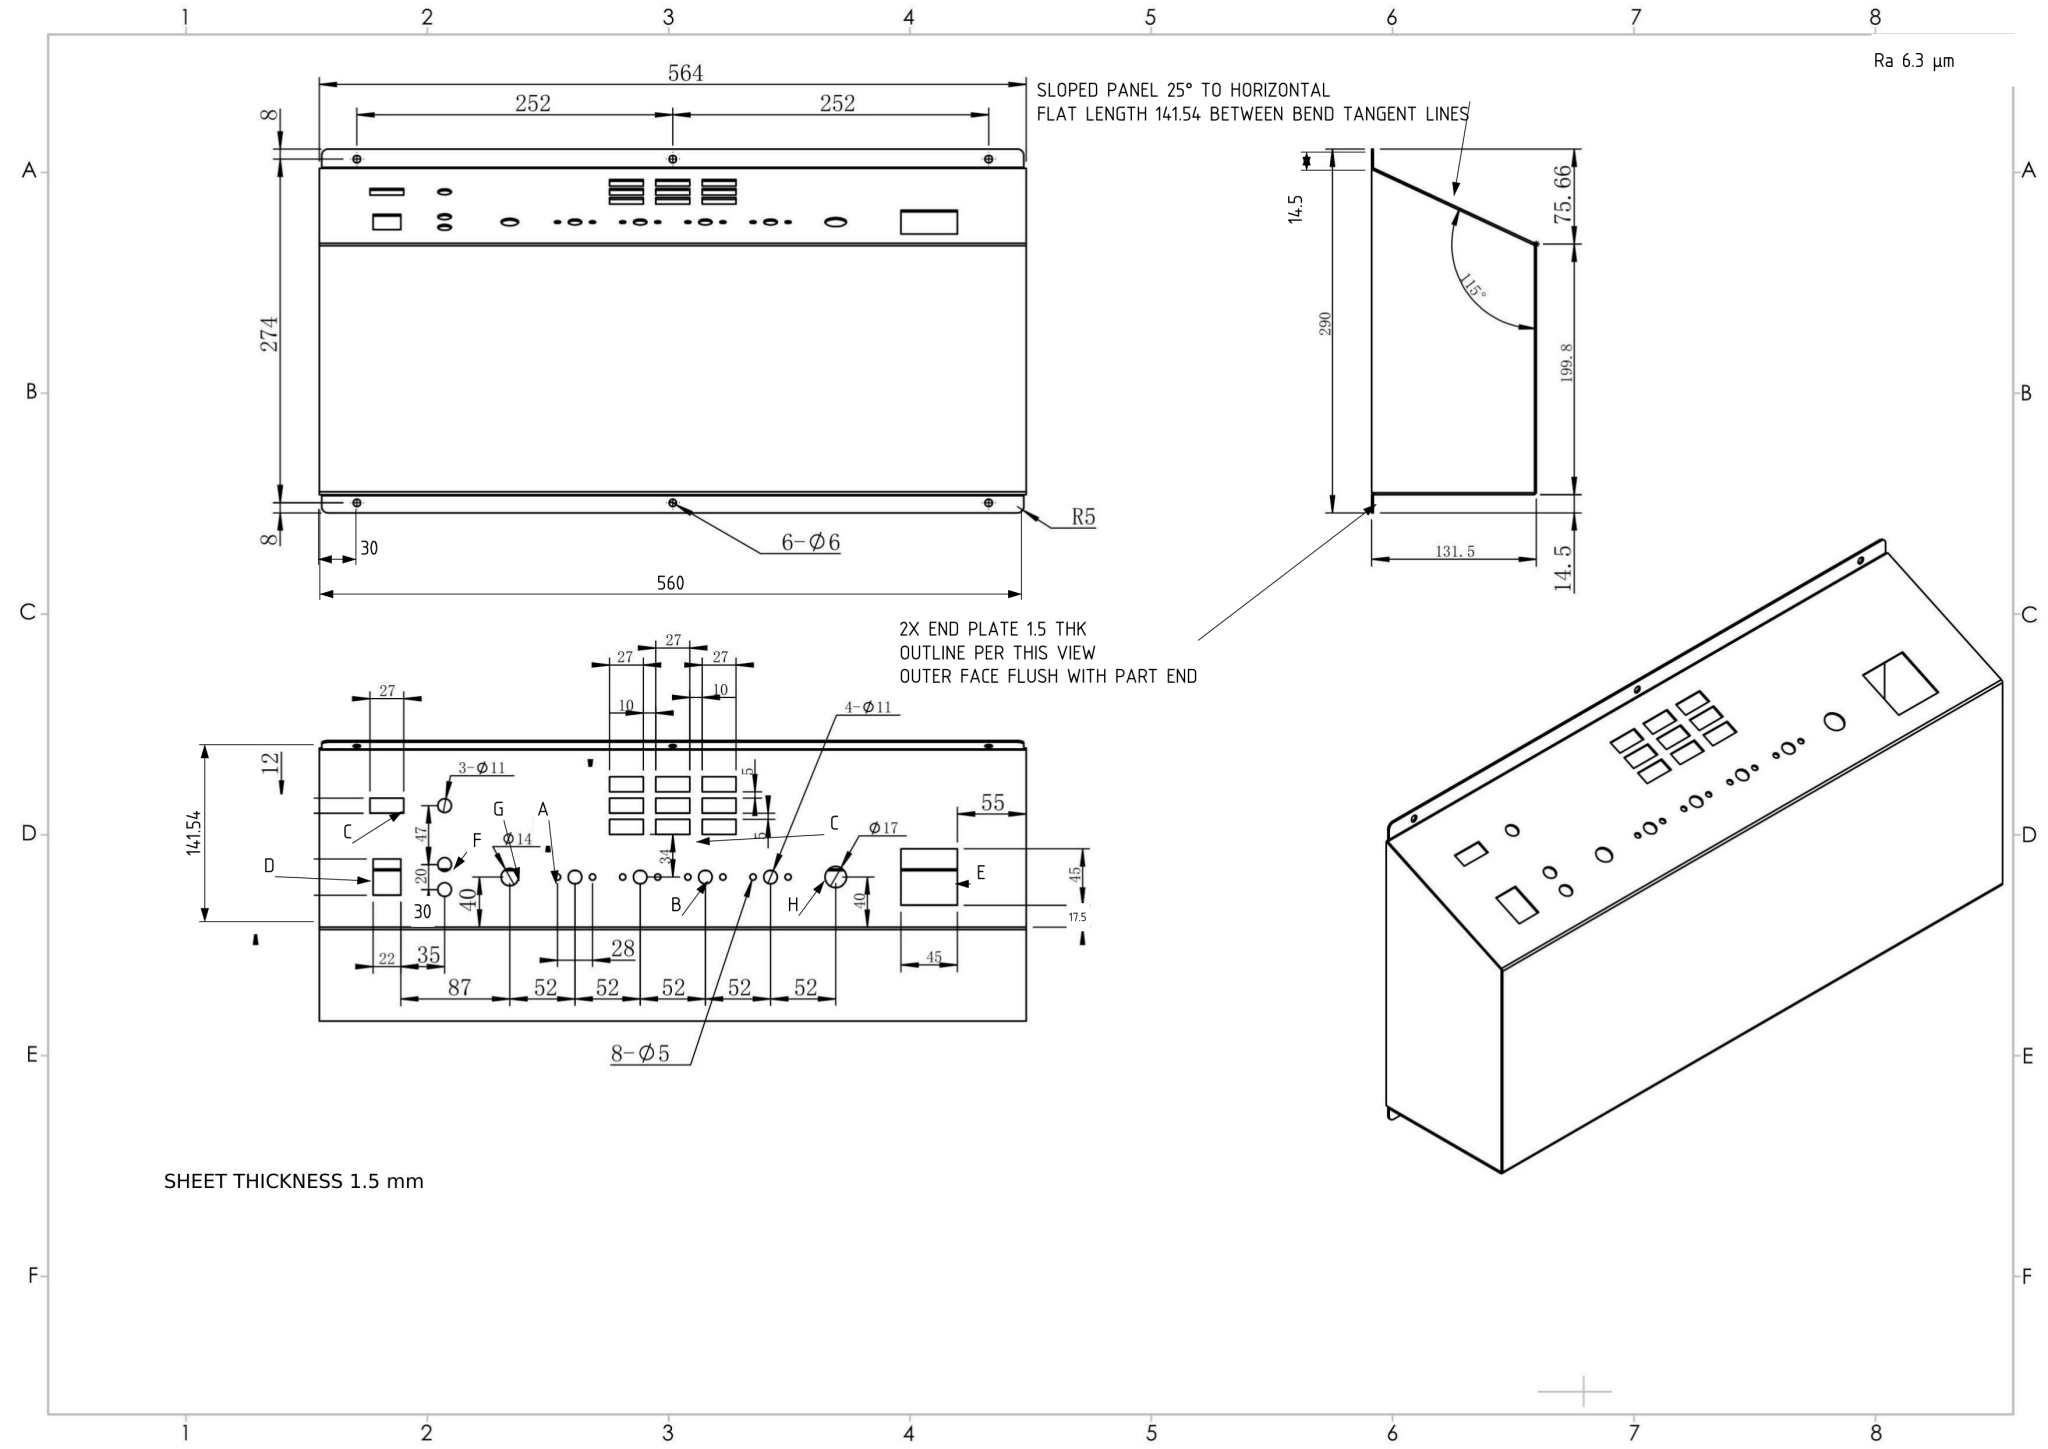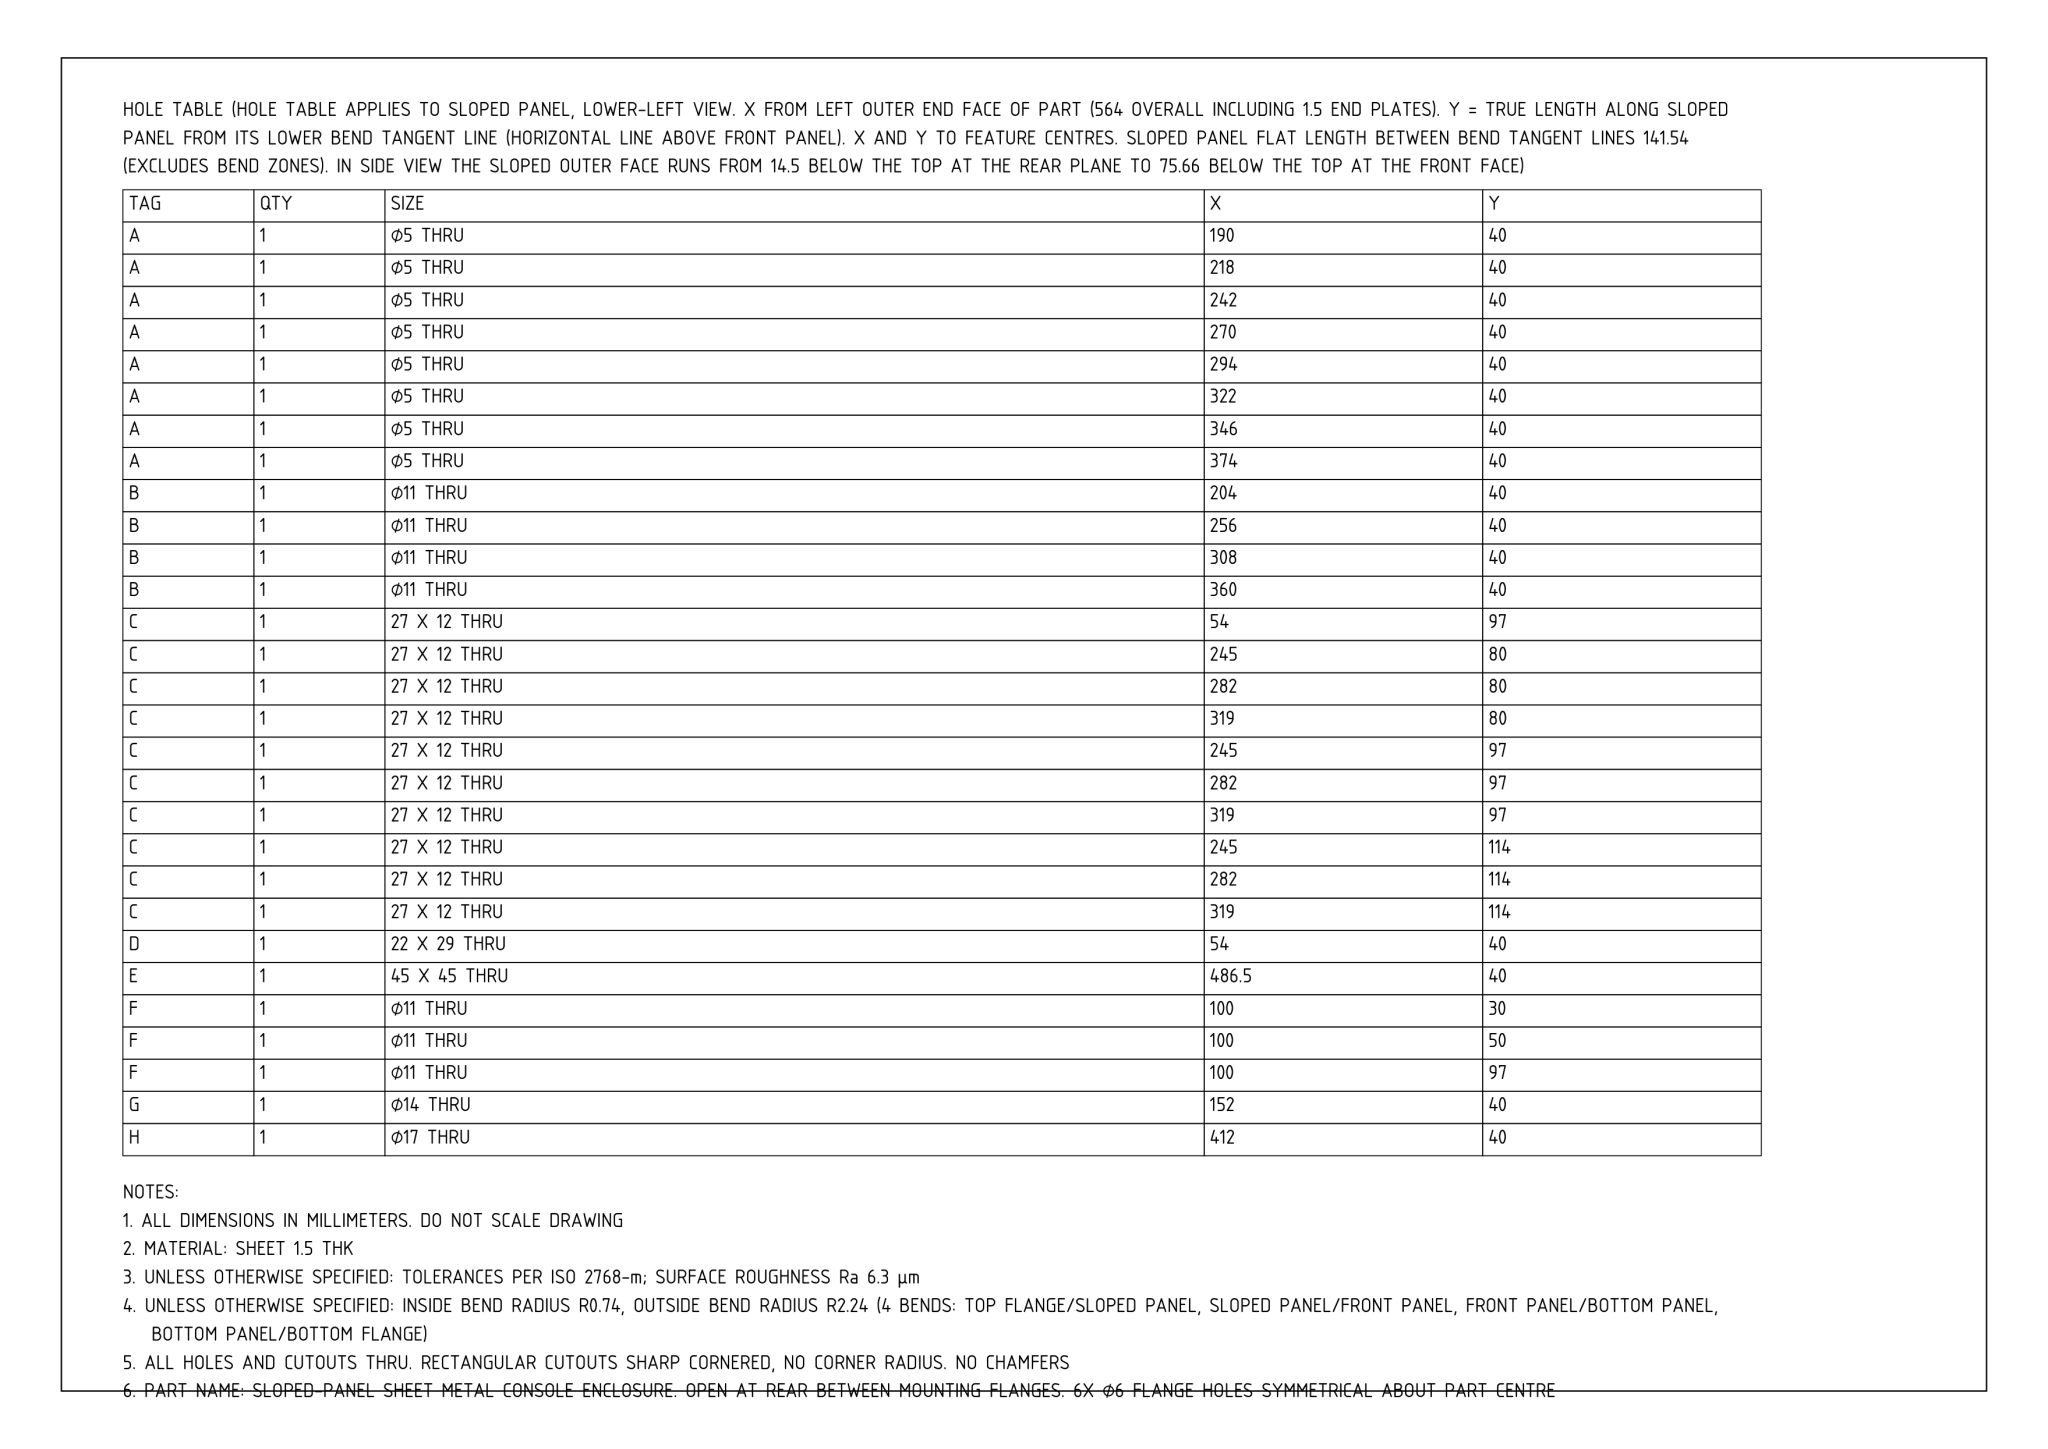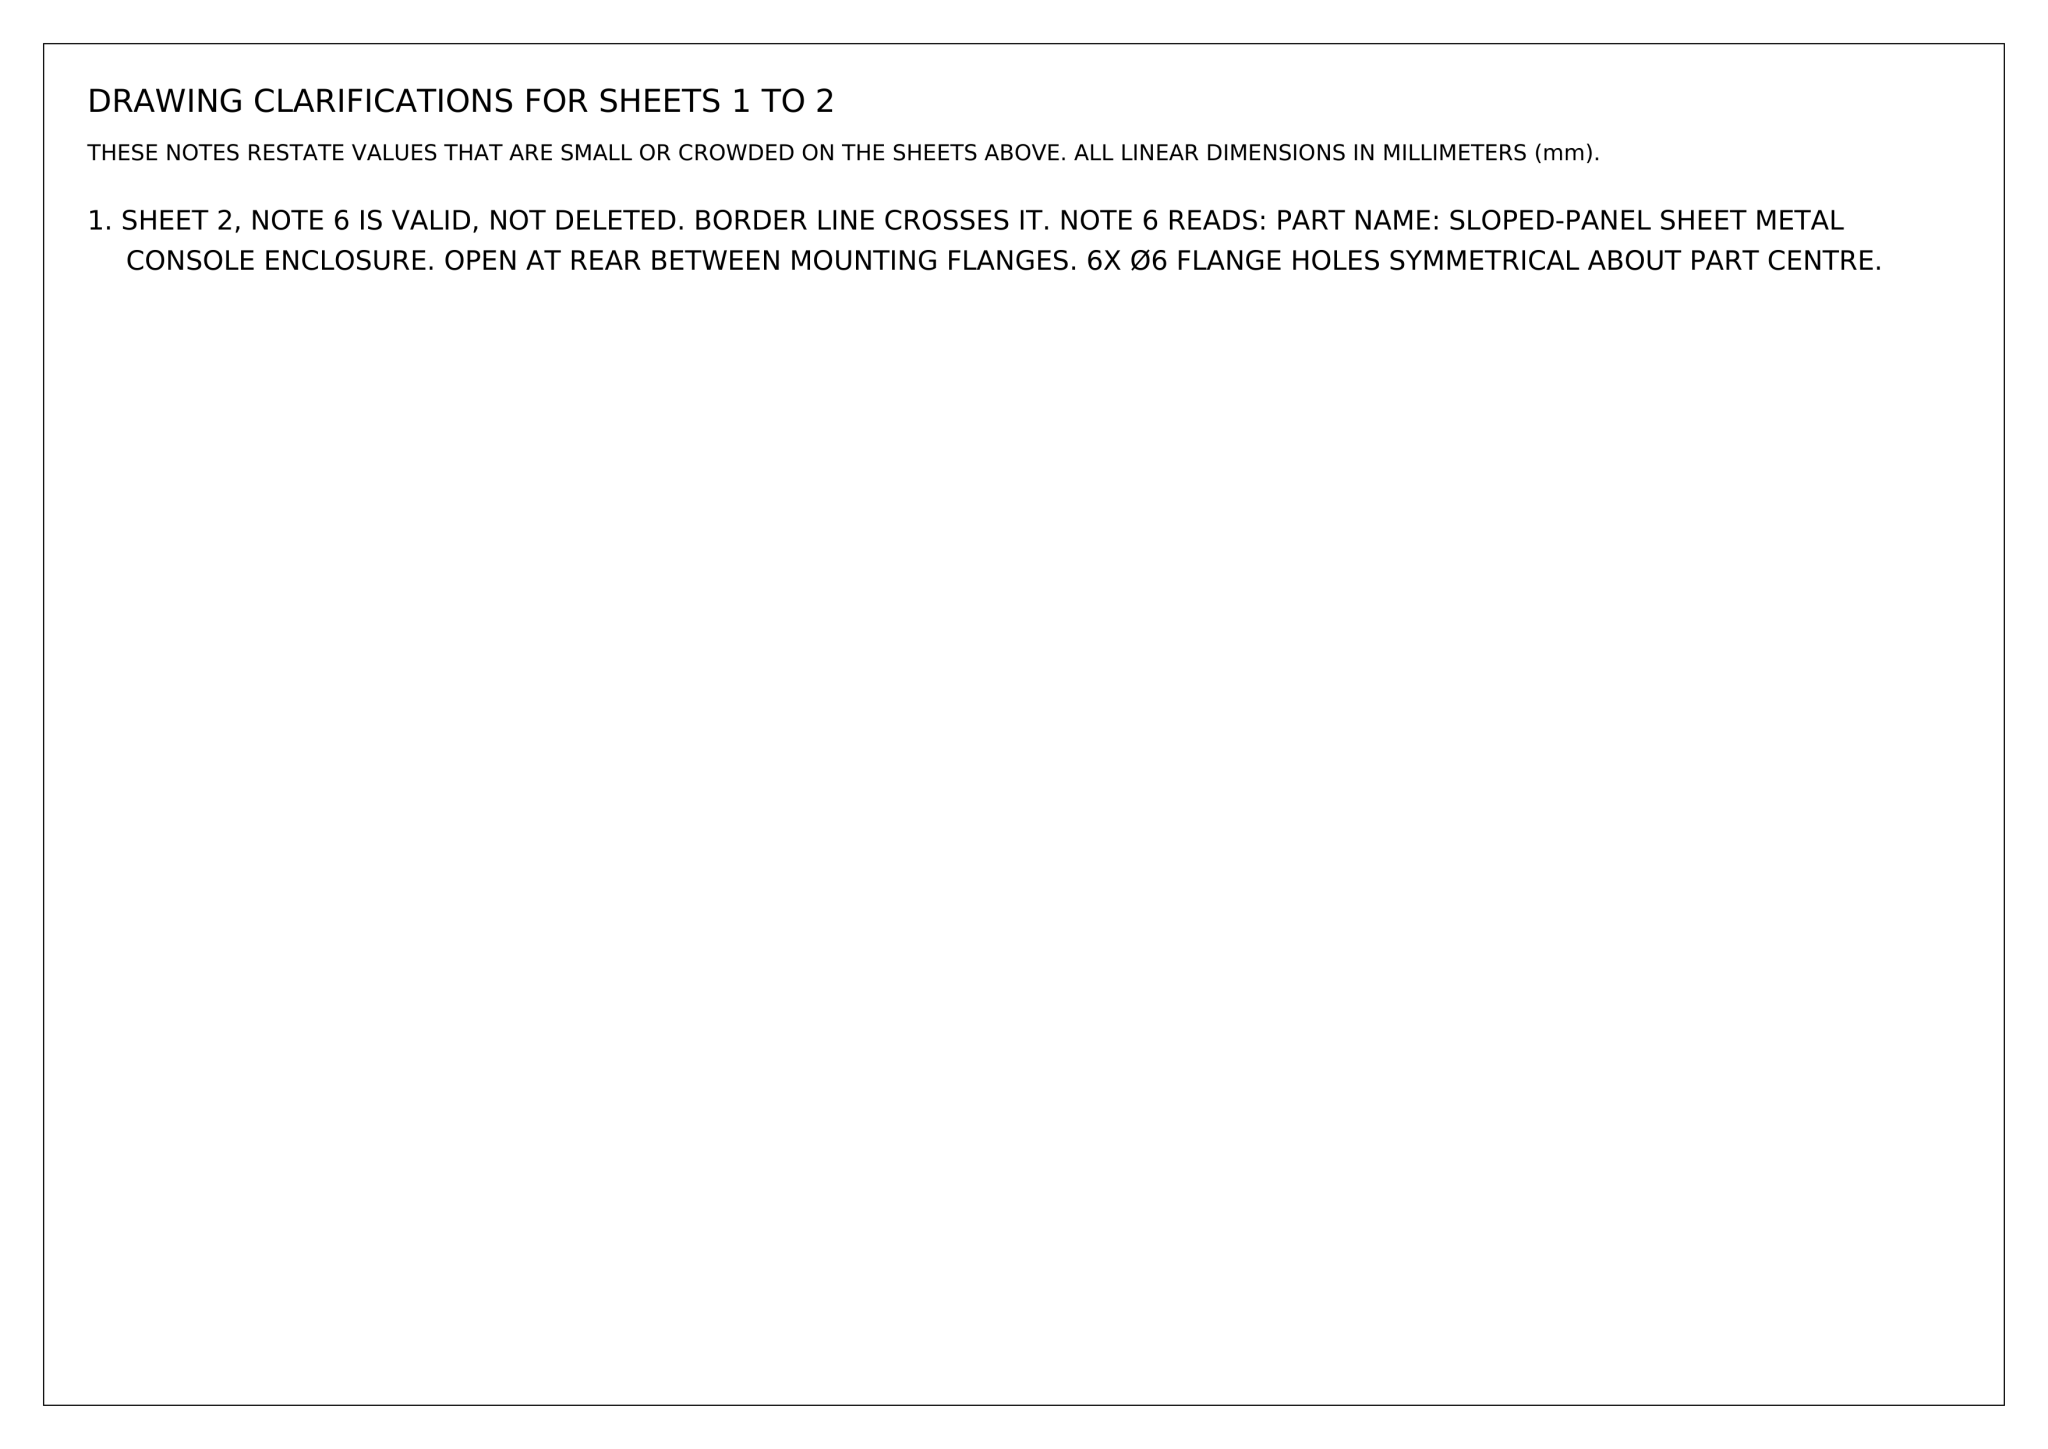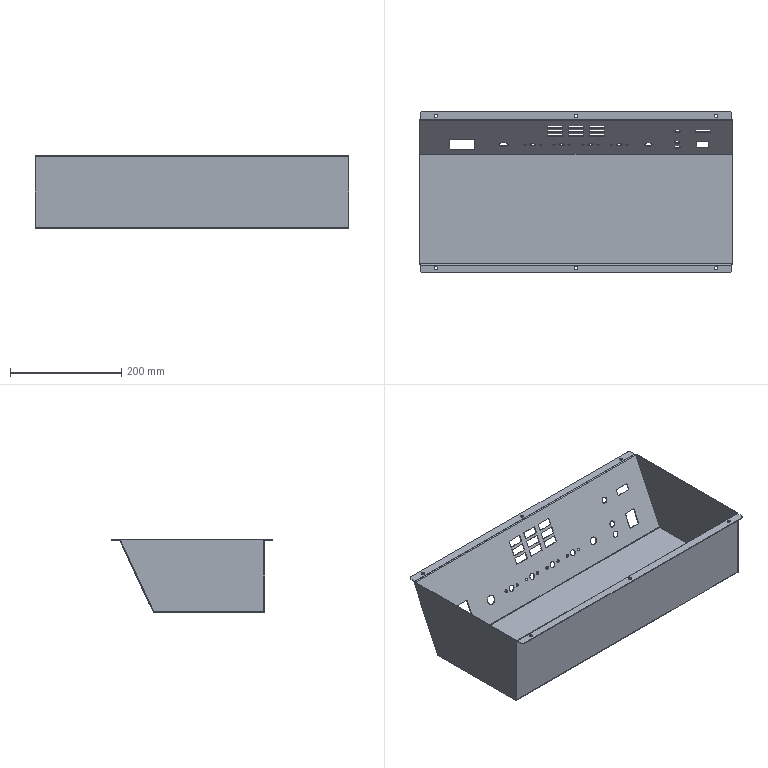Part | NX | mm | 1 solid | 136 faces | box 564 x 290 x 131.5 mm | volume 501613 mm3 | plane 78 | cylinder 58 | commonest cylinder face diameters 5 x16 11 x14 6 x12 1.473 x4 10 x4 4.473 x4 17 x2 14 x2